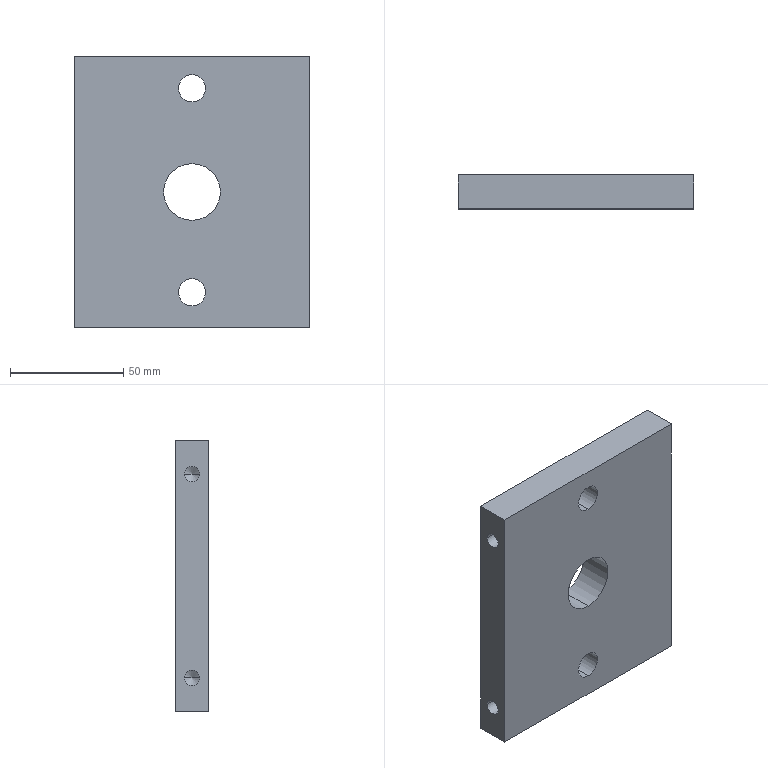Component | SolidWorks | ZL-11-07CrossBeamPlate-1 | 1 solid | 28 faces | box 104 x 15 x 120 mm | volume 173476 mm3 | cylinder 14 | cone 8 | plane 6 | commonest cylinder face diameters 6.8 x8 12 x4 25 x2
build123d program:
from build123d import *

# Parameters (mm, degrees)
SKETCH1_W                  = 120
SKETCH1_H                  = 104
EXTRUDE1_DEPTH             = 7.5
M8_TAPPED_HOLE1_AT_2_COUNT = 2
M8_TAPPED_HOLE1_AT_2_PITCH = 90
M12_TAPPED_HOLE1_D         = 12
F_25_0_25_DIAMETER_HOLE1_D = 25


with BuildPart() as part:
    # Sketch1 → Extrude1 (new, symmetric)
    with BuildSketch(Plane.XY):
        Rectangle(SKETCH1_W, SKETCH1_H)
    extrude(amount=EXTRUDE1_DEPTH, both=True)

    # Sketch3 → M8 Tapped Hole1 (revolve, cut)
    with BuildSketch(Plane(origin=(45, -52, 0), x_dir=(0, 0, -1), z_dir=(1, 0, 0))):
        Polygon((0, 0), (0, 21.793), (3.4, 19.75), (3.4, 0), align=None)
    m8_tapped_hole1 = revolve(axis=Axis((45, -58.35, 0), (0, 1, 0)), mode=Mode.SUBTRACT)

    # M8 Tapped Hole1 at 2: M8 Tapped Hole1 ×2
    with Locations(*[(-i * M8_TAPPED_HOLE1_AT_2_PITCH, 0, 0) for i in range(1, M8_TAPPED_HOLE1_AT_2_COUNT)]):
        add(m8_tapped_hole1, mode=Mode.SUBTRACT)

    # Mirror1: M8 Tapped Hole1 across plane
    add(m8_tapped_hole1.mirror(Plane.ZX), mode=Mode.SUBTRACT)

    # Mirror1 copy 1 sketch → Mirror1 copy 1 (revolve, cut)
    with BuildSketch(Plane(origin=(-45, 52, 0), x_dir=(0, 0, -1), z_dir=(1, 0, 0))):
        Polygon((0, 0), (0, -21.793), (3.4, -19.75), (3.4, 0), align=None)
    revolve(axis=Axis((-45, 58.35, 0), (0, 1, 0)), mode=Mode.SUBTRACT)

    # M12 Tapped Hole1 (through all)
    with Locations(Plane(origin=(44.232, 0, 7.5), x_dir=(1, 0, 0), z_dir=(0, 0, 1))):
        with Locations((0, 0), (-90, 0)):
            Hole(M12_TAPPED_HOLE1_D / 2)

    # 25.0 _25_ Diameter Hole1 (through all)
    with Locations(Plane.XY.offset(7.5)):
        with Locations((0, 0)):
            Hole(F_25_0_25_DIAMETER_HOLE1_D / 2)


solid = part.part

# Placed as in the assembly
solid = solid.moved(Location((125.552, 241.72, 0), (90, 0, -90)))
STEP:
#1=COLOUR_RGB('',0.7922,0.8196,0.9333);
#2=FILL_AREA_STYLE_COLOUR('',#1);
#3=FILL_AREA_STYLE('',(#2));
#4=SURFACE_STYLE_FILL_AREA(#3);
#5=SURFACE_SIDE_STYLE('',(#4));
#6=SURFACE_STYLE_USAGE(.BOTH.,#5);
#7=PRESENTATION_STYLE_ASSIGNMENT((#6));
#8=CARTESIAN_POINT('',(4.943,9.812,0.4921));
#9=VERTEX_POINT('',#8);
#10=CARTESIAN_POINT('',(4.943,9.812,-0.4921));
#11=VERTEX_POINT('',#10);
#12=CARTESIAN_POINT('',(4.943,9.812,-0.));
#13=DIRECTION('',(-0.,-1.,-0.));
#14=DIRECTION('',(0.,0.,-1.));
#15=AXIS2_PLACEMENT_3D('',#12,#13,#14);
#16=CIRCLE('',#15,0.4921);
#17=EDGE_CURVE('',#9,#11,#16,.T.);
#18=ORIENTED_EDGE('',*,*,#17,.F.);
#19=CARTESIAN_POINT('',(4.943,9.221,0.4921));
#20=VERTEX_POINT('',#19);
#21=CARTESIAN_POINT('',(4.943,9.221,0.4921));
#22=DIRECTION('',(-0.,-1.,-0.));
#23=VECTOR('',#22,39.37);
#24=LINE('',#21,#23);
#25=EDGE_CURVE('',#9,#20,#24,.T.);
#26=ORIENTED_EDGE('',*,*,#25,.T.);
#27=CARTESIAN_POINT('',(4.943,9.221,-0.4921));
#28=VERTEX_POINT('',#27);
#29=CARTESIAN_POINT('',(4.943,9.221,-0.));
#30=DIRECTION('',(-0.,-1.,-0.));
#31=DIRECTION('',(0.,0.,-1.));
#32=AXIS2_PLACEMENT_3D('',#29,#30,#31);
#33=CIRCLE('',#32,0.4921);
#34=EDGE_CURVE('',#20,#28,#33,.T.);
#35=ORIENTED_EDGE('',*,*,#34,.T.);
#36=CARTESIAN_POINT('',(4.943,9.221,-0.4921));
#37=DIRECTION('',(-0.,-1.,-0.));
#38=VECTOR('',#37,39.37);
#39=LINE('',#36,#38);
#40=EDGE_CURVE('',#11,#28,#39,.T.);
#41=ORIENTED_EDGE('',*,*,#40,.F.);
#42=EDGE_LOOP('',(#18,#26,#35,#41));
#43=FACE_OUTER_BOUND('',#42,.T.);
#44=CARTESIAN_POINT('',(4.943,9.221,-0.));
#45=DIRECTION('',(-0.,-1.,-0.));
#46=DIRECTION('',(0.,0.,-1.));
#47=AXIS2_PLACEMENT_3D('',#44,#45,#46);
#48=CYLINDRICAL_SURFACE('',#47,0.4921);
#49=ADVANCED_FACE('',(#43),#48,.F.);
#50=CARTESIAN_POINT('',(4.943,9.812,2.038));
#51=VERTEX_POINT('',#50);
#52=CARTESIAN_POINT('',(4.943,9.812,1.566));
#53=VERTEX_POINT('',#52);
#54=CARTESIAN_POINT('',(4.943,9.812,1.802));
#55=DIRECTION('',(-0.,-1.,-0.));
#56=DIRECTION('',(0.,0.,-1.));
#57=AXIS2_PLACEMENT_3D('',#54,#55,#56);
#58=CIRCLE('',#57,0.2362);
#59=EDGE_CURVE('',#51,#53,#58,.T.);
#60=ORIENTED_EDGE('',*,*,#59,.F.);
#61=CARTESIAN_POINT('',(4.943,9.221,2.038));
#62=VERTEX_POINT('',#61);
#63=CARTESIAN_POINT('',(4.943,9.221,2.038));
#64=DIRECTION('',(-0.,-1.,-0.));
#65=VECTOR('',#64,39.37);
#66=LINE('',#63,#65);
#67=EDGE_CURVE('',#51,#62,#66,.T.);
#68=ORIENTED_EDGE('',*,*,#67,.T.);
#69=CARTESIAN_POINT('',(4.943,9.221,1.566));
#70=VERTEX_POINT('',#69);
#71=CARTESIAN_POINT('',(4.943,9.221,1.802));
#72=DIRECTION('',(-0.,-1.,-0.));
#73=DIRECTION('',(0.,0.,-1.));
#74=AXIS2_PLACEMENT_3D('',#71,#72,#73);
#75=CIRCLE('',#74,0.2362);
#76=EDGE_CURVE('',#62,#70,#75,.T.);
#77=ORIENTED_EDGE('',*,*,#76,.T.);
#78=CARTESIAN_POINT('',(4.943,9.221,1.566));
#79=DIRECTION('',(-0.,-1.,-0.));
#80=VECTOR('',#79,39.37);
#81=LINE('',#78,#80);
#82=EDGE_CURVE('',#53,#70,#81,.T.);
#83=ORIENTED_EDGE('',*,*,#82,.F.);
#84=EDGE_LOOP('',(#60,#68,#77,#83));
#85=FACE_OUTER_BOUND('',#84,.T.);
#86=CARTESIAN_POINT('',(4.943,9.221,1.802));
#87=DIRECTION('',(-0.,-1.,-0.));
#88=DIRECTION('',(0.,0.,-1.));
#89=AXIS2_PLACEMENT_3D('',#86,#87,#88);
#90=CYLINDRICAL_SURFACE('',#89,0.2362);
#91=ADVANCED_FACE('',(#85),#90,.F.);
#92=CARTESIAN_POINT('',(4.943,9.812,-1.505));
#93=VERTEX_POINT('',#92);
#94=CARTESIAN_POINT('',(4.943,9.812,-1.978));
#95=VERTEX_POINT('',#94);
#96=CARTESIAN_POINT('',(4.943,9.812,-1.741));
#97=DIRECTION('',(-0.,-1.,-0.));
#98=DIRECTION('',(0.,0.,-1.));
#99=AXIS2_PLACEMENT_3D('',#96,#97,#98);
#100=CIRCLE('',#99,0.2362);
#101=EDGE_CURVE('',#93,#95,#100,.T.);
#102=ORIENTED_EDGE('',*,*,#101,.F.);
#103=CARTESIAN_POINT('',(4.943,9.221,-1.505));
#104=VERTEX_POINT('',#103);
#105=CARTESIAN_POINT('',(4.943,9.221,-1.505));
#106=DIRECTION('',(-0.,-1.,-0.));
#107=VECTOR('',#106,39.37);
#108=LINE('',#105,#107);
#109=EDGE_CURVE('',#93,#104,#108,.T.);
#110=ORIENTED_EDGE('',*,*,#109,.T.);
#111=CARTESIAN_POINT('',(4.943,9.221,-1.978));
#112=VERTEX_POINT('',#111);
#113=CARTESIAN_POINT('',(4.943,9.221,-1.741));
#114=DIRECTION('',(-0.,-1.,-0.));
#115=DIRECTION('',(0.,0.,-1.));
#116=AXIS2_PLACEMENT_3D('',#113,#114,#115);
#117=CIRCLE('',#116,0.2362);
#118=EDGE_CURVE('',#104,#112,#117,.T.);
#119=ORIENTED_EDGE('',*,*,#118,.T.);
#120=CARTESIAN_POINT('',(4.943,9.221,-1.978));
#121=DIRECTION('',(-0.,-1.,-0.));
#122=VECTOR('',#121,39.37);
#123=LINE('',#120,#122);
#124=EDGE_CURVE('',#95,#112,#123,.T.);
#125=ORIENTED_EDGE('',*,*,#124,.F.);
#126=EDGE_LOOP('',(#102,#110,#119,#125));
#127=FACE_OUTER_BOUND('',#126,.T.);
#128=CARTESIAN_POINT('',(4.943,9.221,-1.741));
#129=DIRECTION('',(-0.,-1.,-0.));
#130=DIRECTION('',(0.,0.,-1.));
#131=AXIS2_PLACEMENT_3D('',#128,#129,#130);
#132=CYLINDRICAL_SURFACE('',#131,0.2362);
#133=ADVANCED_FACE('',(#127),#132,.F.);
#134=CARTESIAN_POINT('',(6.132,9.517,1.772));
#135=VERTEX_POINT('',#134);
#136=CARTESIAN_POINT('',(6.213,9.383,1.772));
#137=VERTEX_POINT('',#136);
#138=CARTESIAN_POINT('',(6.213,9.383,1.772));
#139=DIRECTION('',(0.515,-0.8572,-0.));
#140=VECTOR('',#139,39.37);
#141=LINE('',#138,#140);
#142=EDGE_CURVE('',#135,#137,#141,.T.);
#143=ORIENTED_EDGE('',*,*,#142,.F.);
#144=CARTESIAN_POINT('',(6.213,9.65,1.772));
#145=VERTEX_POINT('',#144);
#146=CARTESIAN_POINT('',(6.213,9.65,1.772));
#147=DIRECTION('',(0.515,0.8572,0.));
#148=VECTOR('',#147,39.37);
#149=LINE('',#146,#148);
#150=EDGE_CURVE('',#135,#145,#149,.T.);
#151=ORIENTED_EDGE('',*,*,#150,.T.);
#152=CARTESIAN_POINT('',(6.213,9.517,1.772));
#153=DIRECTION('',(1.,-0.,-0.));
#154=DIRECTION('',(0.,-1.,0.));
#155=AXIS2_PLACEMENT_3D('',#152,#153,#154);
#156=CIRCLE('',#155,0.1339);
#157=EDGE_CURVE('',#145,#137,#156,.T.);
#158=ORIENTED_EDGE('',*,*,#157,.T.);
#159=EDGE_LOOP('',(#143,#151,#158));
#160=FACE_OUTER_BOUND('',#159,.T.);
#161=CARTESIAN_POINT('',(6.213,9.517,1.772));
#162=DIRECTION('',(1.,-0.,-0.));
#163=DIRECTION('',(0.,-1.,0.));
#164=AXIS2_PLACEMENT_3D('',#161,#162,#163);
#165=CONICAL_SURFACE('',#164,0.1339,1.03);
#166=ADVANCED_FACE('',(#160),#165,.F.);
#167=ORIENTED_EDGE('',*,*,#157,.F.);
#168=CARTESIAN_POINT('',(6.99,9.65,1.772));
#169=VERTEX_POINT('',#168);
#170=CARTESIAN_POINT('',(6.99,9.65,1.772));
#171=DIRECTION('',(1.,-0.,-0.));
#172=VECTOR('',#171,39.37);
#173=LINE('',#170,#172);
#174=EDGE_CURVE('',#145,#169,#173,.T.);
#175=ORIENTED_EDGE('',*,*,#174,.T.);
#176=CARTESIAN_POINT('',(6.99,9.383,1.772));
#177=VERTEX_POINT('',#176);
#178=CARTESIAN_POINT('',(6.99,9.517,1.772));
#179=DIRECTION('',(1.,-0.,-0.));
#180=DIRECTION('',(0.,-1.,0.));
#181=AXIS2_PLACEMENT_3D('',#178,#179,#180);
#182=CIRCLE('',#181,0.1339);
#183=EDGE_CURVE('',#169,#177,#182,.T.);
#184=ORIENTED_EDGE('',*,*,#183,.T.);
#185=CARTESIAN_POINT('',(6.99,9.383,1.772));
#186=DIRECTION('',(1.,-0.,-0.));
#187=VECTOR('',#186,39.37);
#188=LINE('',#185,#187);
#189=EDGE_CURVE('',#137,#177,#188,.T.);
#190=ORIENTED_EDGE('',*,*,#189,.F.);
#191=EDGE_LOOP('',(#167,#175,#184,#190));
#192=FACE_OUTER_BOUND('',#191,.T.);
#193=CARTESIAN_POINT('',(6.99,9.517,1.772));
#194=DIRECTION('',(1.,-0.,-0.));
#195=DIRECTION('',(0.,-1.,0.));
#196=AXIS2_PLACEMENT_3D('',#193,#194,#195);
#197=CYLINDRICAL_SURFACE('',#196,0.1339);
#198=ADVANCED_FACE('',(#192),#197,.F.);
#199=CARTESIAN_POINT('',(6.132,9.517,-1.772));
#200=VERTEX_POINT('',#199);
#201=CARTESIAN_POINT('',(6.213,9.383,-1.772));
#202=VERTEX_POINT('',#201);
#203=CARTESIAN_POINT('',(6.213,9.383,-1.772));
#204=DIRECTION('',(0.515,-0.8572,-0.));
#205=VECTOR('',#204,39.37);
#206=LINE('',#203,#205);
#207=EDGE_CURVE('',#200,#202,#206,.T.);
#208=ORIENTED_EDGE('',*,*,#207,.F.);
#209=CARTESIAN_POINT('',(6.213,9.65,-1.772));
#210=VERTEX_POINT('',#209);
#211=CARTESIAN_POINT('',(6.213,9.65,-1.772));
#212=DIRECTION('',(0.515,0.8572,0.));
#213=VECTOR('',#212,39.37);
#214=LINE('',#211,#213);
#215=EDGE_CURVE('',#200,#210,#214,.T.);
#216=ORIENTED_EDGE('',*,*,#215,.T.);
#217=CARTESIAN_POINT('',(6.213,9.517,-1.772));
#218=DIRECTION('',(1.,-0.,-0.));
#219=DIRECTION('',(0.,-1.,0.));
#220=AXIS2_PLACEMENT_3D('',#217,#218,#219);
#221=CIRCLE('',#220,0.1339);
#222=EDGE_CURVE('',#210,#202,#221,.T.);
#223=ORIENTED_EDGE('',*,*,#222,.T.);
#224=EDGE_LOOP('',(#208,#216,#223));
#225=FACE_OUTER_BOUND('',#224,.T.);
#226=CARTESIAN_POINT('',(6.213,9.517,-1.772));
#227=DIRECTION('',(1.,-0.,-0.));
#228=DIRECTION('',(0.,-1.,0.));
#229=AXIS2_PLACEMENT_3D('',#226,#227,#228);
#230=CONICAL_SURFACE('',#229,0.1339,1.03);
#231=ADVANCED_FACE('',(#225),#230,.F.);
#232=ORIENTED_EDGE('',*,*,#222,.F.);
#233=CARTESIAN_POINT('',(6.99,9.65,-1.772));
#234=VERTEX_POINT('',#233);
#235=CARTESIAN_POINT('',(6.99,9.65,-1.772));
#236=DIRECTION('',(1.,-0.,-0.));
#237=VECTOR('',#236,39.37);
#238=LINE('',#235,#237);
#239=EDGE_CURVE('',#210,#234,#238,.T.);
#240=ORIENTED_EDGE('',*,*,#239,.T.);
#241=CARTESIAN_POINT('',(6.99,9.383,-1.772));
#242=VERTEX_POINT('',#241);
#243=CARTESIAN_POINT('',(6.99,9.517,-1.772));
#244=DIRECTION('',(1.,-0.,-0.));
#245=DIRECTION('',(0.,-1.,0.));
#246=AXIS2_PLACEMENT_3D('',#243,#244,#245);
#247=CIRCLE('',#246,0.1339);
#248=EDGE_CURVE('',#234,#242,#247,.T.);
#249=ORIENTED_EDGE('',*,*,#248,.T.);
#250=CARTESIAN_POINT('',(6.99,9.383,-1.772));
#251=DIRECTION('',(1.,-0.,-0.));
#252=VECTOR('',#251,39.37);
#253=LINE('',#250,#252);
#254=EDGE_CURVE('',#202,#242,#253,.T.);
#255=ORIENTED_EDGE('',*,*,#254,.F.);
#256=EDGE_LOOP('',(#232,#240,#249,#255));
#257=FACE_OUTER_BOUND('',#256,.T.);
#258=CARTESIAN_POINT('',(6.99,9.517,-1.772));
#259=DIRECTION('',(1.,-0.,-0.));
#260=DIRECTION('',(0.,-1.,0.));
#261=AXIS2_PLACEMENT_3D('',#258,#259,#260);
#262=CYLINDRICAL_SURFACE('',#261,0.1339);
#263=ADVANCED_FACE('',(#257),#262,.F.);
#264=CARTESIAN_POINT('',(3.754,9.517,1.772));
#265=VERTEX_POINT('',#264);
#266=CARTESIAN_POINT('',(3.673,9.65,1.772));
#267=VERTEX_POINT('',#266);
#268=CARTESIAN_POINT('',(3.673,9.65,1.772));
#269=DIRECTION('',(-0.515,0.8572,0.));
#270=VECTOR('',#269,39.37);
#271=LINE('',#268,#270);
#272=EDGE_CURVE('',#265,#267,#271,.T.);
#273=ORIENTED_EDGE('',*,*,#272,.F.);
#274=CARTESIAN_POINT('',(3.673,9.383,1.772));
#275=VERTEX_POINT('',#274);
#276=CARTESIAN_POINT('',(3.673,9.383,1.772));
#277=DIRECTION('',(-0.515,-0.8572,-0.));
#278=VECTOR('',#277,39.37);
#279=LINE('',#276,#278);
#280=EDGE_CURVE('',#265,#275,#279,.T.);
#281=ORIENTED_EDGE('',*,*,#280,.T.);
#282=CARTESIAN_POINT('',(3.673,9.517,1.772));
#283=DIRECTION('',(-1.,0.,0.));
#284=DIRECTION('',(0.,1.,0.));
#285=AXIS2_PLACEMENT_3D('',#282,#283,#284);
#286=CIRCLE('',#285,0.1339);
#287=EDGE_CURVE('',#275,#267,#286,.T.);
#288=ORIENTED_EDGE('',*,*,#287,.T.);
#289=EDGE_LOOP('',(#273,#281,#288));
#290=FACE_OUTER_BOUND('',#289,.T.);
#291=CARTESIAN_POINT('',(3.673,9.517,1.772));
#292=DIRECTION('',(-1.,0.,0.));
#293=DIRECTION('',(0.,1.,0.));
#294=AXIS2_PLACEMENT_3D('',#291,#292,#293);
#295=CONICAL_SURFACE('',#294,0.1339,1.03);
#296=ADVANCED_FACE('',(#290),#295,.F.);
#297=ORIENTED_EDGE('',*,*,#287,.F.);
#298=CARTESIAN_POINT('',(2.896,9.383,1.772));
#299=VERTEX_POINT('',#298);
#300=CARTESIAN_POINT('',(2.896,9.383,1.772));
#301=DIRECTION('',(-1.,0.,0.));
#302=VECTOR('',#301,39.37);
#303=LINE('',#300,#302);
#304=EDGE_CURVE('',#275,#299,#303,.T.);
#305=ORIENTED_EDGE('',*,*,#304,.T.);
#306=CARTESIAN_POINT('',(2.896,9.65,1.772));
#307=VERTEX_POINT('',#306);
#308=CARTESIAN_POINT('',(2.896,9.517,1.772));
#309=DIRECTION('',(-1.,0.,0.));
#310=DIRECTION('',(0.,1.,0.));
#311=AXIS2_PLACEMENT_3D('',#308,#309,#310);
#312=CIRCLE('',#311,0.1339);
#313=EDGE_CURVE('',#299,#307,#312,.T.);
#314=ORIENTED_EDGE('',*,*,#313,.T.);
#315=CARTESIAN_POINT('',(2.896,9.65,1.772));
#316=DIRECTION('',(-1.,0.,0.));
#317=VECTOR('',#316,39.37);
#318=LINE('',#315,#317);
#319=EDGE_CURVE('',#267,#307,#318,.T.);
#320=ORIENTED_EDGE('',*,*,#319,.F.);
#321=EDGE_LOOP('',(#297,#305,#314,#320));
#322=FACE_OUTER_BOUND('',#321,.T.);
#323=CARTESIAN_POINT('',(2.896,9.517,1.772));
#324=DIRECTION('',(-1.,0.,0.));
#325=DIRECTION('',(0.,1.,0.));
#326=AXIS2_PLACEMENT_3D('',#323,#324,#325);
#327=CYLINDRICAL_SURFACE('',#326,0.1339);
#328=ADVANCED_FACE('',(#322),#327,.F.);
#329=CARTESIAN_POINT('',(3.754,9.517,-1.772));
#330=VERTEX_POINT('',#329);
#331=CARTESIAN_POINT('',(3.673,9.65,-1.772));
#332=VERTEX_POINT('',#331);
#333=CARTESIAN_POINT('',(3.673,9.65,-1.772));
#334=DIRECTION('',(-0.515,0.8572,0.));
#335=VECTOR('',#334,39.37);
#336=LINE('',#333,#335);
#337=EDGE_CURVE('',#330,#332,#336,.T.);
#338=ORIENTED_EDGE('',*,*,#337,.F.);
#339=CARTESIAN_POINT('',(3.673,9.383,-1.772));
#340=VERTEX_POINT('',#339);
#341=CARTESIAN_POINT('',(3.673,9.383,-1.772));
#342=DIRECTION('',(-0.515,-0.8572,-0.));
#343=VECTOR('',#342,39.37);
#344=LINE('',#341,#343);
#345=EDGE_CURVE('',#330,#340,#344,.T.);
#346=ORIENTED_EDGE('',*,*,#345,.T.);
#347=CARTESIAN_POINT('',(3.673,9.517,-1.772));
#348=DIRECTION('',(-1.,0.,0.));
#349=DIRECTION('',(0.,1.,0.));
#350=AXIS2_PLACEMENT_3D('',#347,#348,#349);
#351=CIRCLE('',#350,0.1339);
#352=EDGE_CURVE('',#340,#332,#351,.T.);
#353=ORIENTED_EDGE('',*,*,#352,.T.);
#354=EDGE_LOOP('',(#338,#346,#353));
#355=FACE_OUTER_BOUND('',#354,.T.);
#356=CARTESIAN_POINT('',(3.673,9.517,-1.772));
#357=DIRECTION('',(-1.,0.,0.));
#358=DIRECTION('',(0.,1.,0.));
#359=AXIS2_PLACEMENT_3D('',#356,#357,#358);
#360=CONICAL_SURFACE('',#359,0.1339,1.03);
#361=ADVANCED_FACE('',(#355),#360,.F.);
#362=ORIENTED_EDGE('',*,*,#352,.F.);
#363=CARTESIAN_POINT('',(2.896,9.383,-1.772));
#364=VERTEX_POINT('',#363);
#365=CARTESIAN_POINT('',(2.896,9.383,-1.772));
#366=DIRECTION('',(-1.,0.,0.));
#367=VECTOR('',#366,39.37);
#368=LINE('',#365,#367);
#369=EDGE_CURVE('',#340,#364,#368,.T.);
#370=ORIENTED_EDGE('',*,*,#369,.T.);
#371=CARTESIAN_POINT('',(2.896,9.65,-1.772));
#372=VERTEX_POINT('',#371);
#373=CARTESIAN_POINT('',(2.896,9.517,-1.772));
#374=DIRECTION('',(-1.,0.,0.));
#375=DIRECTION('',(0.,1.,0.));
#376=AXIS2_PLACEMENT_3D('',#373,#374,#375);
#377=CIRCLE('',#376,0.1339);
#378=EDGE_CURVE('',#364,#372,#377,.T.);
#379=ORIENTED_EDGE('',*,*,#378,.T.);
#380=CARTESIAN_POINT('',(2.896,9.65,-1.772));
#381=DIRECTION('',(-1.,0.,0.));
#382=VECTOR('',#381,39.37);
#383=LINE('',#380,#382);
#384=EDGE_CURVE('',#332,#372,#383,.T.);
#385=ORIENTED_EDGE('',*,*,#384,.F.);
#386=EDGE_LOOP('',(#362,#370,#379,#385));
#387=FACE_OUTER_BOUND('',#386,.T.);
#388=CARTESIAN_POINT('',(2.896,9.517,-1.772));
#389=DIRECTION('',(-1.,0.,0.));
#390=DIRECTION('',(0.,1.,0.));
#391=AXIS2_PLACEMENT_3D('',#388,#389,#390);
#392=CYLINDRICAL_SURFACE('',#391,0.1339);
#393=ADVANCED_FACE('',(#387),#392,.F.);
#394=CARTESIAN_POINT('',(6.99,9.812,2.362));
#395=VERTEX_POINT('',#394);
#396=CARTESIAN_POINT('',(2.896,9.812,2.362));
#397=VERTEX_POINT('',#396);
#398=CARTESIAN_POINT('',(6.99,9.812,2.362));
#399=DIRECTION('',(-1.,0.,0.));
#400=VECTOR('',#399,39.37);
#401=LINE('',#398,#400);
#402=EDGE_CURVE('',#395,#397,#401,.T.);
#403=ORIENTED_EDGE('',*,*,#402,.T.);
#404=CARTESIAN_POINT('',(2.896,9.221,2.362));
#405=VERTEX_POINT('',#404);
#406=CARTESIAN_POINT('',(2.896,9.221,2.362));
#407=DIRECTION('',(0.,1.,0.));
#408=VECTOR('',#407,39.37);
#409=LINE('',#406,#408);
#410=EDGE_CURVE('',#405,#397,#409,.T.);
#411=ORIENTED_EDGE('',*,*,#410,.F.);
#412=CARTESIAN_POINT('',(6.99,9.221,2.362));
#413=VERTEX_POINT('',#412);
#414=CARTESIAN_POINT('',(6.99,9.221,2.362));
#415=DIRECTION('',(-1.,0.,0.));
#416=VECTOR('',#415,39.37);
#417=LINE('',#414,#416);
#418=EDGE_CURVE('',#413,#405,#417,.T.);
#419=ORIENTED_EDGE('',*,*,#418,.F.);
#420=CARTESIAN_POINT('',(6.99,9.221,2.362));
#421=DIRECTION('',(0.,1.,0.));
#422=VECTOR('',#421,39.37);
#423=LINE('',#420,#422);
#424=EDGE_CURVE('',#413,#395,#423,.T.);
#425=ORIENTED_EDGE('',*,*,#424,.T.);
#426=EDGE_LOOP('',(#403,#411,#419,#425));
#427=FACE_OUTER_BOUND('',#426,.T.);
#428=CARTESIAN_POINT('',(6.99,9.221,2.362));
#429=DIRECTION('',(-0.,0.,-1.));
#430=DIRECTION('',(0.,1.,0.));
#431=AXIS2_PLACEMENT_3D('',#428,#429,#430);
#432=PLANE('',#431);
#433=ADVANCED_FACE('',(#427),#432,.F.);
#434=CARTESIAN_POINT('',(2.896,9.517,1.772));
#435=DIRECTION('',(-1.,0.,0.));
#436=DIRECTION('',(0.,1.,0.));
#437=AXIS2_PLACEMENT_3D('',#434,#435,#436);
#438=CIRCLE('',#437,0.1339);
#439=EDGE_CURVE('',#307,#299,#438,.T.);
#440=ORIENTED_EDGE('',*,*,#439,.F.);
#441=ORIENTED_EDGE('',*,*,#313,.F.);
#442=EDGE_LOOP('',(#440,#441));
#443=FACE_BOUND('',#442,.T.);
#444=CARTESIAN_POINT('',(2.896,9.517,-1.772));
#445=DIRECTION('',(-1.,0.,0.));
#446=DIRECTION('',(0.,1.,0.));
#447=AXIS2_PLACEMENT_3D('',#444,#445,#446);
#448=CIRCLE('',#447,0.1339);
#449=EDGE_CURVE('',#372,#364,#448,.T.);
#450=ORIENTED_EDGE('',*,*,#449,.F.);
#451=ORIENTED_EDGE('',*,*,#378,.F.);
#452=EDGE_LOOP('',(#450,#451));
#453=FACE_BOUND('',#452,.T.);
#454=CARTESIAN_POINT('',(2.896,9.812,-2.362));
#455=VERTEX_POINT('',#454);
#456=CARTESIAN_POINT('',(2.896,9.812,2.362));
#457=DIRECTION('',(-0.,0.,-1.));
#458=VECTOR('',#457,39.37);
#459=LINE('',#456,#458);
#460=EDGE_CURVE('',#397,#455,#459,.T.);
#461=ORIENTED_EDGE('',*,*,#460,.T.);
#462=CARTESIAN_POINT('',(2.896,9.221,-2.362));
#463=VERTEX_POINT('',#462);
#464=CARTESIAN_POINT('',(2.896,9.221,-2.362));
#465=DIRECTION('',(0.,1.,0.));
#466=VECTOR('',#465,39.37);
#467=LINE('',#464,#466);
#468=EDGE_CURVE('',#463,#455,#467,.T.);
#469=ORIENTED_EDGE('',*,*,#468,.F.);
#470=CARTESIAN_POINT('',(2.896,9.221,2.362));
#471=DIRECTION('',(-0.,0.,-1.));
#472=VECTOR('',#471,39.37);
#473=LINE('',#470,#472);
#474=EDGE_CURVE('',#405,#463,#473,.T.);
#475=ORIENTED_EDGE('',*,*,#474,.F.);
#476=ORIENTED_EDGE('',*,*,#410,.T.);
#477=EDGE_LOOP('',(#461,#469,#475,#476));
#478=FACE_OUTER_BOUND('',#477,.T.);
#479=CARTESIAN_POINT('',(2.896,9.221,2.362));
#480=DIRECTION('',(1.,-0.,-0.));
#481=DIRECTION('',(-0.,-1.,-0.));
#482=AXIS2_PLACEMENT_3D('',#479,#480,#481);
#483=PLANE('',#482);
#484=ADVANCED_FACE('',(#443,#453,#478),#483,.F.);
#485=CARTESIAN_POINT('',(6.99,9.812,-2.362));
#486=VERTEX_POINT('',#485);
#487=CARTESIAN_POINT('',(6.99,9.812,-2.362));
#488=DIRECTION('',(1.,-0.,-0.));
#489=VECTOR('',#488,39.37);
#490=LINE('',#487,#489);
#491=EDGE_CURVE('',#455,#486,#490,.T.);
#492=ORIENTED_EDGE('',*,*,#491,.T.);
#493=CARTESIAN_POINT('',(6.99,9.221,-2.362));
#494=VERTEX_POINT('',#493);
#495=CARTESIAN_POINT('',(6.99,9.221,-2.362));
#496=DIRECTION('',(0.,1.,0.));
#497=VECTOR('',#496,39.37);
#498=LINE('',#495,#497);
#499=EDGE_CURVE('',#494,#486,#498,.T.);
#500=ORIENTED_EDGE('',*,*,#499,.F.);
#501=CARTESIAN_POINT('',(6.99,9.221,-2.362));
#502=DIRECTION('',(1.,-0.,-0.));
#503=VECTOR('',#502,39.37);
#504=LINE('',#501,#503);
#505=EDGE_CURVE('',#463,#494,#504,.T.);
#506=ORIENTED_EDGE('',*,*,#505,.F.);
#507=ORIENTED_EDGE('',*,*,#468,.T.);
#508=EDGE_LOOP('',(#492,#500,#506,#507));
#509=FACE_OUTER_BOUND('',#508,.T.);
#510=CARTESIAN_POINT('',(6.99,9.221,-2.362));
#511=DIRECTION('',(0.,-0.,1.));
#512=DIRECTION('',(-0.,-1.,-0.));
#513=AXIS2_PLACEMENT_3D('',#510,#511,#512);
#514=PLANE('',#513);
#515=ADVANCED_FACE('',(#509),#514,.F.);
#516=CARTESIAN_POINT('',(6.99,9.517,1.772));
#517=DIRECTION('',(1.,-0.,-0.));
#518=DIRECTION('',(0.,-1.,0.));
#519=AXIS2_PLACEMENT_3D('',#516,#517,#518);
#520=CIRCLE('',#519,0.1339);
#521=EDGE_CURVE('',#177,#169,#520,.T.);
#522=ORIENTED_EDGE('',*,*,#521,.F.);
#523=ORIENTED_EDGE('',*,*,#183,.F.);
#524=EDGE_LOOP('',(#522,#523));
#525=FACE_BOUND('',#524,.T.);
#526=CARTESIAN_POINT('',(6.99,9.517,-1.772));
#527=DIRECTION('',(1.,-0.,-0.));
#528=DIRECTION('',(0.,-1.,0.));
#529=AXIS2_PLACEMENT_3D('',#526,#527,#528);
#530=CIRCLE('',#529,0.1339);
#531=EDGE_CURVE('',#242,#234,#530,.T.);
#532=ORIENTED_EDGE('',*,*,#531,.F.);
#533=ORIENTED_EDGE('',*,*,#248,.F.);
#534=EDGE_LOOP('',(#532,#533));
#535=FACE_BOUND('',#534,.T.);
#536=CARTESIAN_POINT('',(6.99,9.812,2.362));
#537=DIRECTION('',(0.,-0.,1.));
#538=VECTOR('',#537,39.37);
#539=LINE('',#536,#538);
#540=EDGE_CURVE('',#486,#395,#539,.T.);
#541=ORIENTED_EDGE('',*,*,#540,.T.);
#542=ORIENTED_EDGE('',*,*,#424,.F.);
#543=CARTESIAN_POINT('',(6.99,9.221,2.362));
#544=DIRECTION('',(0.,-0.,1.));
#545=VECTOR('',#544,39.37);
#546=LINE('',#543,#545);
#547=EDGE_CURVE('',#494,#413,#546,.T.);
#548=ORIENTED_EDGE('',*,*,#547,.F.);
#549=ORIENTED_EDGE('',*,*,#499,.T.);
#550=EDGE_LOOP('',(#541,#542,#548,#549));
#551=FACE_OUTER_BOUND('',#550,.T.);
#552=CARTESIAN_POINT('',(6.99,9.221,2.362));
#553=DIRECTION('',(-1.,0.,0.));
#554=DIRECTION('',(-0.,0.,-1.));
#555=AXIS2_PLACEMENT_3D('',#552,#553,#554);
#556=PLANE('',#555);
#557=ADVANCED_FACE('',(#525,#535,#551),#556,.F.);
#558=CARTESIAN_POINT('',(4.943,9.221,-0.));
#559=DIRECTION('',(-0.,-1.,-0.));
#560=DIRECTION('',(0.,0.,-1.));
#561=AXIS2_PLACEMENT_3D('',#558,#559,#560);
#562=CIRCLE('',#561,0.4921);
#563=EDGE_CURVE('',#28,#20,#562,.T.);
#564=ORIENTED_EDGE('',*,*,#563,.F.);
#565=ORIENTED_EDGE('',*,*,#34,.F.);
#566=EDGE_LOOP('',(#564,#565));
#567=FACE_BOUND('',#566,.T.);
#568=CARTESIAN_POINT('',(4.943,9.221,1.802));
#569=DIRECTION('',(-0.,-1.,-0.));
#570=DIRECTION('',(0.,0.,-1.));
#571=AXIS2_PLACEMENT_3D('',#568,#569,#570);
#572=CIRCLE('',#571,0.2362);
#573=EDGE_CURVE('',#70,#62,#572,.T.);
#574=ORIENTED_EDGE('',*,*,#573,.F.);
#575=ORIENTED_EDGE('',*,*,#76,.F.);
#576=EDGE_LOOP('',(#574,#575));
#577=FACE_BOUND('',#576,.T.);
#578=CARTESIAN_POINT('',(4.943,9.221,-1.741));
#579=DIRECTION('',(-0.,-1.,-0.));
#580=DIRECTION('',(0.,0.,-1.));
#581=AXIS2_PLACEMENT_3D('',#578,#579,#580);
#582=CIRCLE('',#581,0.2362);
#583=EDGE_CURVE('',#112,#104,#582,.T.);
#584=ORIENTED_EDGE('',*,*,#583,.F.);
#585=ORIENTED_EDGE('',*,*,#118,.F.);
#586=EDGE_LOOP('',(#584,#585));
#587=FACE_BOUND('',#586,.T.);
#588=ORIENTED_EDGE('',*,*,#418,.T.);
#589=ORIENTED_EDGE('',*,*,#474,.T.);
#590=ORIENTED_EDGE('',*,*,#505,.T.);
#591=ORIENTED_EDGE('',*,*,#547,.T.);
#592=EDGE_LOOP('',(#588,#589,#590,#591));
#593=FACE_OUTER_BOUND('',#592,.T.);
#594=CARTESIAN_POINT('',(2.896,9.221,2.362));
#595=DIRECTION('',(-0.,-1.,-0.));
#596=DIRECTION('',(-0.,0.,-1.));
#597=AXIS2_PLACEMENT_3D('',#594,#595,#596);
#598=PLANE('',#597);
#599=ADVANCED_FACE('',(#567,#577,#587,#593),#598,.T.);
#600=CARTESIAN_POINT('',(4.943,9.812,-0.));
#601=DIRECTION('',(-0.,-1.,-0.));
#602=DIRECTION('',(0.,0.,-1.));
#603=AXIS2_PLACEMENT_3D('',#600,#601,#602);
#604=CIRCLE('',#603,0.4921);
#605=EDGE_CURVE('',#11,#9,#604,.T.);
#606=ORIENTED_EDGE('',*,*,#605,.T.);
#607=ORIENTED_EDGE('',*,*,#17,.T.);
#608=EDGE_LOOP('',(#606,#607));
#609=FACE_BOUND('',#608,.T.);
#610=CARTESIAN_POINT('',(4.943,9.812,1.802));
#611=DIRECTION('',(-0.,-1.,-0.));
#612=DIRECTION('',(0.,0.,-1.));
#613=AXIS2_PLACEMENT_3D('',#610,#611,#612);
#614=CIRCLE('',#613,0.2362);
#615=EDGE_CURVE('',#53,#51,#614,.T.);
#616=ORIENTED_EDGE('',*,*,#615,.T.);
#617=ORIENTED_EDGE('',*,*,#59,.T.);
#618=EDGE_LOOP('',(#616,#617));
#619=FACE_BOUND('',#618,.T.);
#620=CARTESIAN_POINT('',(4.943,9.812,-1.741));
#621=DIRECTION('',(-0.,-1.,-0.));
#622=DIRECTION('',(0.,0.,-1.));
#623=AXIS2_PLACEMENT_3D('',#620,#621,#622);
#624=CIRCLE('',#623,0.2362);
#625=EDGE_CURVE('',#95,#93,#624,.T.);
#626=ORIENTED_EDGE('',*,*,#625,.T.);
#627=ORIENTED_EDGE('',*,*,#101,.T.);
#628=EDGE_LOOP('',(#626,#627));
#629=FACE_BOUND('',#628,.T.);
#630=ORIENTED_EDGE('',*,*,#402,.F.);
#631=ORIENTED_EDGE('',*,*,#540,.F.);
#632=ORIENTED_EDGE('',*,*,#491,.F.);
#633=ORIENTED_EDGE('',*,*,#460,.F.);
#634=EDGE_LOOP('',(#630,#631,#632,#633));
#635=FACE_OUTER_BOUND('',#634,.T.);
#636=CARTESIAN_POINT('',(2.896,9.812,2.362));
#637=DIRECTION('',(-0.,-1.,-0.));
#638=DIRECTION('',(-0.,0.,-1.));
#639=AXIS2_PLACEMENT_3D('',#636,#637,#638);
#640=PLANE('',#639);
#641=ADVANCED_FACE('',(#609,#619,#629,#635),#640,.F.);
#642=ORIENTED_EDGE('',*,*,#369,.F.);
#643=CARTESIAN_POINT('',(3.673,9.517,-1.772));
#644=DIRECTION('',(-1.,0.,0.));
#645=DIRECTION('',(0.,1.,0.));
#646=AXIS2_PLACEMENT_3D('',#643,#644,#645);
#647=CIRCLE('',#646,0.1339);
#648=EDGE_CURVE('',#332,#340,#647,.T.);
#649=ORIENTED_EDGE('',*,*,#648,.F.);
#650=ORIENTED_EDGE('',*,*,#384,.T.);
#651=ORIENTED_EDGE('',*,*,#449,.T.);
#652=EDGE_LOOP('',(#642,#649,#650,#651));
#653=FACE_OUTER_BOUND('',#652,.T.);
#654=CARTESIAN_POINT('',(2.896,9.517,-1.772));
#655=DIRECTION('',(-1.,0.,0.));
#656=DIRECTION('',(0.,1.,0.));
#657=AXIS2_PLACEMENT_3D('',#654,#655,#656);
#658=CYLINDRICAL_SURFACE('',#657,0.1339);
#659=ADVANCED_FACE('',(#653),#658,.F.);
#660=ORIENTED_EDGE('',*,*,#345,.F.);
#661=ORIENTED_EDGE('',*,*,#337,.T.);
#662=ORIENTED_EDGE('',*,*,#648,.T.);
#663=EDGE_LOOP('',(#660,#661,#662));
#664=FACE_OUTER_BOUND('',#663,.T.);
#665=CARTESIAN_POINT('',(3.673,9.517,-1.772));
#666=DIRECTION('',(-1.,0.,0.));
#667=DIRECTION('',(0.,1.,0.));
#668=AXIS2_PLACEMENT_3D('',#665,#666,#667);
#669=CONICAL_SURFACE('',#668,0.1339,1.03);
#670=ADVANCED_FACE('',(#664),#669,.F.);
#671=ORIENTED_EDGE('',*,*,#304,.F.);
#672=CARTESIAN_POINT('',(3.673,9.517,1.772));
#673=DIRECTION('',(-1.,0.,0.));
#674=DIRECTION('',(0.,1.,0.));
#675=AXIS2_PLACEMENT_3D('',#672,#673,#674);
#676=CIRCLE('',#675,0.1339);
#677=EDGE_CURVE('',#267,#275,#676,.T.);
#678=ORIENTED_EDGE('',*,*,#677,.F.);
#679=ORIENTED_EDGE('',*,*,#319,.T.);
#680=ORIENTED_EDGE('',*,*,#439,.T.);
#681=EDGE_LOOP('',(#671,#678,#679,#680));
#682=FACE_OUTER_BOUND('',#681,.T.);
#683=CARTESIAN_POINT('',(2.896,9.517,1.772));
#684=DIRECTION('',(-1.,0.,0.));
#685=DIRECTION('',(0.,1.,0.));
#686=AXIS2_PLACEMENT_3D('',#683,#684,#685);
#687=CYLINDRICAL_SURFACE('',#686,0.1339);
#688=ADVANCED_FACE('',(#682),#687,.F.);
#689=ORIENTED_EDGE('',*,*,#280,.F.);
#690=ORIENTED_EDGE('',*,*,#272,.T.);
#691=ORIENTED_EDGE('',*,*,#677,.T.);
#692=EDGE_LOOP('',(#689,#690,#691));
#693=FACE_OUTER_BOUND('',#692,.T.);
#694=CARTESIAN_POINT('',(3.673,9.517,1.772));
#695=DIRECTION('',(-1.,0.,0.));
#696=DIRECTION('',(0.,1.,0.));
#697=AXIS2_PLACEMENT_3D('',#694,#695,#696);
#698=CONICAL_SURFACE('',#697,0.1339,1.03);
#699=ADVANCED_FACE('',(#693),#698,.F.);
#700=ORIENTED_EDGE('',*,*,#239,.F.);
#701=CARTESIAN_POINT('',(6.213,9.517,-1.772));
#702=DIRECTION('',(1.,-0.,-0.));
#703=DIRECTION('',(0.,-1.,0.));
#704=AXIS2_PLACEMENT_3D('',#701,#702,#703);
#705=CIRCLE('',#704,0.1339);
#706=EDGE_CURVE('',#202,#210,#705,.T.);
#707=ORIENTED_EDGE('',*,*,#706,.F.);
#708=ORIENTED_EDGE('',*,*,#254,.T.);
#709=ORIENTED_EDGE('',*,*,#531,.T.);
#710=EDGE_LOOP('',(#700,#707,#708,#709));
#711=FACE_OUTER_BOUND('',#710,.T.);
#712=CARTESIAN_POINT('',(6.99,9.517,-1.772));
#713=DIRECTION('',(1.,-0.,-0.));
#714=DIRECTION('',(0.,-1.,0.));
#715=AXIS2_PLACEMENT_3D('',#712,#713,#714);
#716=CYLINDRICAL_SURFACE('',#715,0.1339);
#717=ADVANCED_FACE('',(#711),#716,.F.);
#718=ORIENTED_EDGE('',*,*,#215,.F.);
#719=ORIENTED_EDGE('',*,*,#207,.T.);
#720=ORIENTED_EDGE('',*,*,#706,.T.);
#721=EDGE_LOOP('',(#718,#719,#720));
#722=FACE_OUTER_BOUND('',#721,.T.);
#723=CARTESIAN_POINT('',(6.213,9.517,-1.772));
#724=DIRECTION('',(1.,-0.,-0.));
#725=DIRECTION('',(0.,-1.,0.));
#726=AXIS2_PLACEMENT_3D('',#723,#724,#725);
#727=CONICAL_SURFACE('',#726,0.1339,1.03);
#728=ADVANCED_FACE('',(#722),#727,.F.);
#729=ORIENTED_EDGE('',*,*,#174,.F.);
#730=CARTESIAN_POINT('',(6.213,9.517,1.772));
#731=DIRECTION('',(1.,-0.,-0.));
#732=DIRECTION('',(0.,-1.,0.));
#733=AXIS2_PLACEMENT_3D('',#730,#731,#732);
#734=CIRCLE('',#733,0.1339);
#735=EDGE_CURVE('',#137,#145,#734,.T.);
#736=ORIENTED_EDGE('',*,*,#735,.F.);
#737=ORIENTED_EDGE('',*,*,#189,.T.);
#738=ORIENTED_EDGE('',*,*,#521,.T.);
#739=EDGE_LOOP('',(#729,#736,#737,#738));
#740=FACE_OUTER_BOUND('',#739,.T.);
#741=CARTESIAN_POINT('',(6.99,9.517,1.772));
#742=DIRECTION('',(1.,-0.,-0.));
#743=DIRECTION('',(0.,-1.,0.));
#744=AXIS2_PLACEMENT_3D('',#741,#742,#743);
#745=CYLINDRICAL_SURFACE('',#744,0.1339);
#746=ADVANCED_FACE('',(#740),#745,.F.);
#747=ORIENTED_EDGE('',*,*,#150,.F.);
#748=ORIENTED_EDGE('',*,*,#142,.T.);
#749=ORIENTED_EDGE('',*,*,#735,.T.);
#750=EDGE_LOOP('',(#747,#748,#749));
#751=FACE_OUTER_BOUND('',#750,.T.);
#752=CARTESIAN_POINT('',(6.213,9.517,1.772));
#753=DIRECTION('',(1.,-0.,-0.));
#754=DIRECTION('',(0.,-1.,0.));
#755=AXIS2_PLACEMENT_3D('',#752,#753,#754);
#756=CONICAL_SURFACE('',#755,0.1339,1.03);
#757=ADVANCED_FACE('',(#751),#756,.F.);
#758=ORIENTED_EDGE('',*,*,#109,.F.);
#759=ORIENTED_EDGE('',*,*,#625,.F.);
#760=ORIENTED_EDGE('',*,*,#124,.T.);
#761=ORIENTED_EDGE('',*,*,#583,.T.);
#762=EDGE_LOOP('',(#758,#759,#760,#761));
#763=FACE_OUTER_BOUND('',#762,.T.);
#764=CARTESIAN_POINT('',(4.943,9.221,-1.741));
#765=DIRECTION('',(-0.,-1.,-0.));
#766=DIRECTION('',(0.,0.,-1.));
#767=AXIS2_PLACEMENT_3D('',#764,#765,#766);
#768=CYLINDRICAL_SURFACE('',#767,0.2362);
#769=ADVANCED_FACE('',(#763),#768,.F.);
#770=ORIENTED_EDGE('',*,*,#67,.F.);
#771=ORIENTED_EDGE('',*,*,#615,.F.);
#772=ORIENTED_EDGE('',*,*,#82,.T.);
#773=ORIENTED_EDGE('',*,*,#573,.T.);
#774=EDGE_LOOP('',(#770,#771,#772,#773));
#775=FACE_OUTER_BOUND('',#774,.T.);
#776=CARTESIAN_POINT('',(4.943,9.221,1.802));
#777=DIRECTION('',(-0.,-1.,-0.));
#778=DIRECTION('',(0.,0.,-1.));
#779=AXIS2_PLACEMENT_3D('',#776,#777,#778);
#780=CYLINDRICAL_SURFACE('',#779,0.2362);
#781=ADVANCED_FACE('',(#775),#780,.F.);
#782=ORIENTED_EDGE('',*,*,#25,.F.);
#783=ORIENTED_EDGE('',*,*,#605,.F.);
#784=ORIENTED_EDGE('',*,*,#40,.T.);
#785=ORIENTED_EDGE('',*,*,#563,.T.);
#786=EDGE_LOOP('',(#782,#783,#784,#785));
#787=FACE_OUTER_BOUND('',#786,.T.);
#788=CARTESIAN_POINT('',(4.943,9.221,-0.));
#789=DIRECTION('',(-0.,-1.,-0.));
#790=DIRECTION('',(0.,0.,-1.));
#791=AXIS2_PLACEMENT_3D('',#788,#789,#790);
#792=CYLINDRICAL_SURFACE('',#791,0.4921);
#793=ADVANCED_FACE('',(#787),#792,.F.);
#794=CLOSED_SHELL('',(#49,#91,#133,#166,#198,#231,#263,#296,#328,#361,#393,#433,#484,#515,#557,#599,#641,#659,#670,#688,#699,#717,#728,#746,#757,#769,#781,#793));
#795=MANIFOLD_SOLID_BREP('',#794);
#796=STYLED_ITEM('',(#7),#795);
#797=(LENGTH_UNIT()NAMED_UNIT(*)SI_UNIT($,.METRE.));
#798=LENGTH_MEASURE_WITH_UNIT(LENGTH_MEASURE(0.0254),#797);
#799=DIMENSIONAL_EXPONENTS(1.,0.,0.,0.,0.,0.,0.);
#800=(CONVERSION_BASED_UNIT('',#798)LENGTH_UNIT()NAMED_UNIT(#799));
#801=UNCERTAINTY_MEASURE_WITH_UNIT(LENGTH_MEASURE(0.00001),#800,'','');
#802=(NAMED_UNIT(*)PLANE_ANGLE_UNIT()SI_UNIT($,.RADIAN.));
#803=(NAMED_UNIT(*)SI_UNIT($,.STERADIAN.)SOLID_ANGLE_UNIT());
#804=(GEOMETRIC_REPRESENTATION_CONTEXT(3)GLOBAL_UNCERTAINTY_ASSIGNED_CONTEXT((#801))GLOBAL_UNIT_ASSIGNED_CONTEXT((#800,#802,#803))REPRESENTATION_CONTEXT('',''));
#805=MECHANICAL_DESIGN_GEOMETRIC_PRESENTATION_REPRESENTATION('',(#796),#804);
#806=CARTESIAN_POINT('',(0.,0.,0.));
#807=DIRECTION('',(0.,0.,1.));
#808=DIRECTION('',(1.,0.,0.));
#809=AXIS2_PLACEMENT_3D('',#806,#807,#808);
#810=(LENGTH_UNIT()NAMED_UNIT(*)SI_UNIT($,.METRE.));
#811=LENGTH_MEASURE_WITH_UNIT(LENGTH_MEASURE(0.0254),#810);
#812=DIMENSIONAL_EXPONENTS(1.,0.,0.,0.,0.,0.,0.);
#813=(CONVERSION_BASED_UNIT('',#811)LENGTH_UNIT()NAMED_UNIT(#812));
#814=UNCERTAINTY_MEASURE_WITH_UNIT(LENGTH_MEASURE(0.00001),#813,'','');
#815=(NAMED_UNIT(*)PLANE_ANGLE_UNIT()SI_UNIT($,.RADIAN.));
#816=(NAMED_UNIT(*)SI_UNIT($,.STERADIAN.)SOLID_ANGLE_UNIT());
#817=(GEOMETRIC_REPRESENTATION_CONTEXT(3)GLOBAL_UNCERTAINTY_ASSIGNED_CONTEXT((#814))GLOBAL_UNIT_ASSIGNED_CONTEXT((#813,#815,#816))REPRESENTATION_CONTEXT('',''));
#818=ADVANCED_BREP_SHAPE_REPRESENTATION('',(#795,#809),#817);
#819=PRESENTATION_LAYER_ASSIGNMENT('','',(#796));